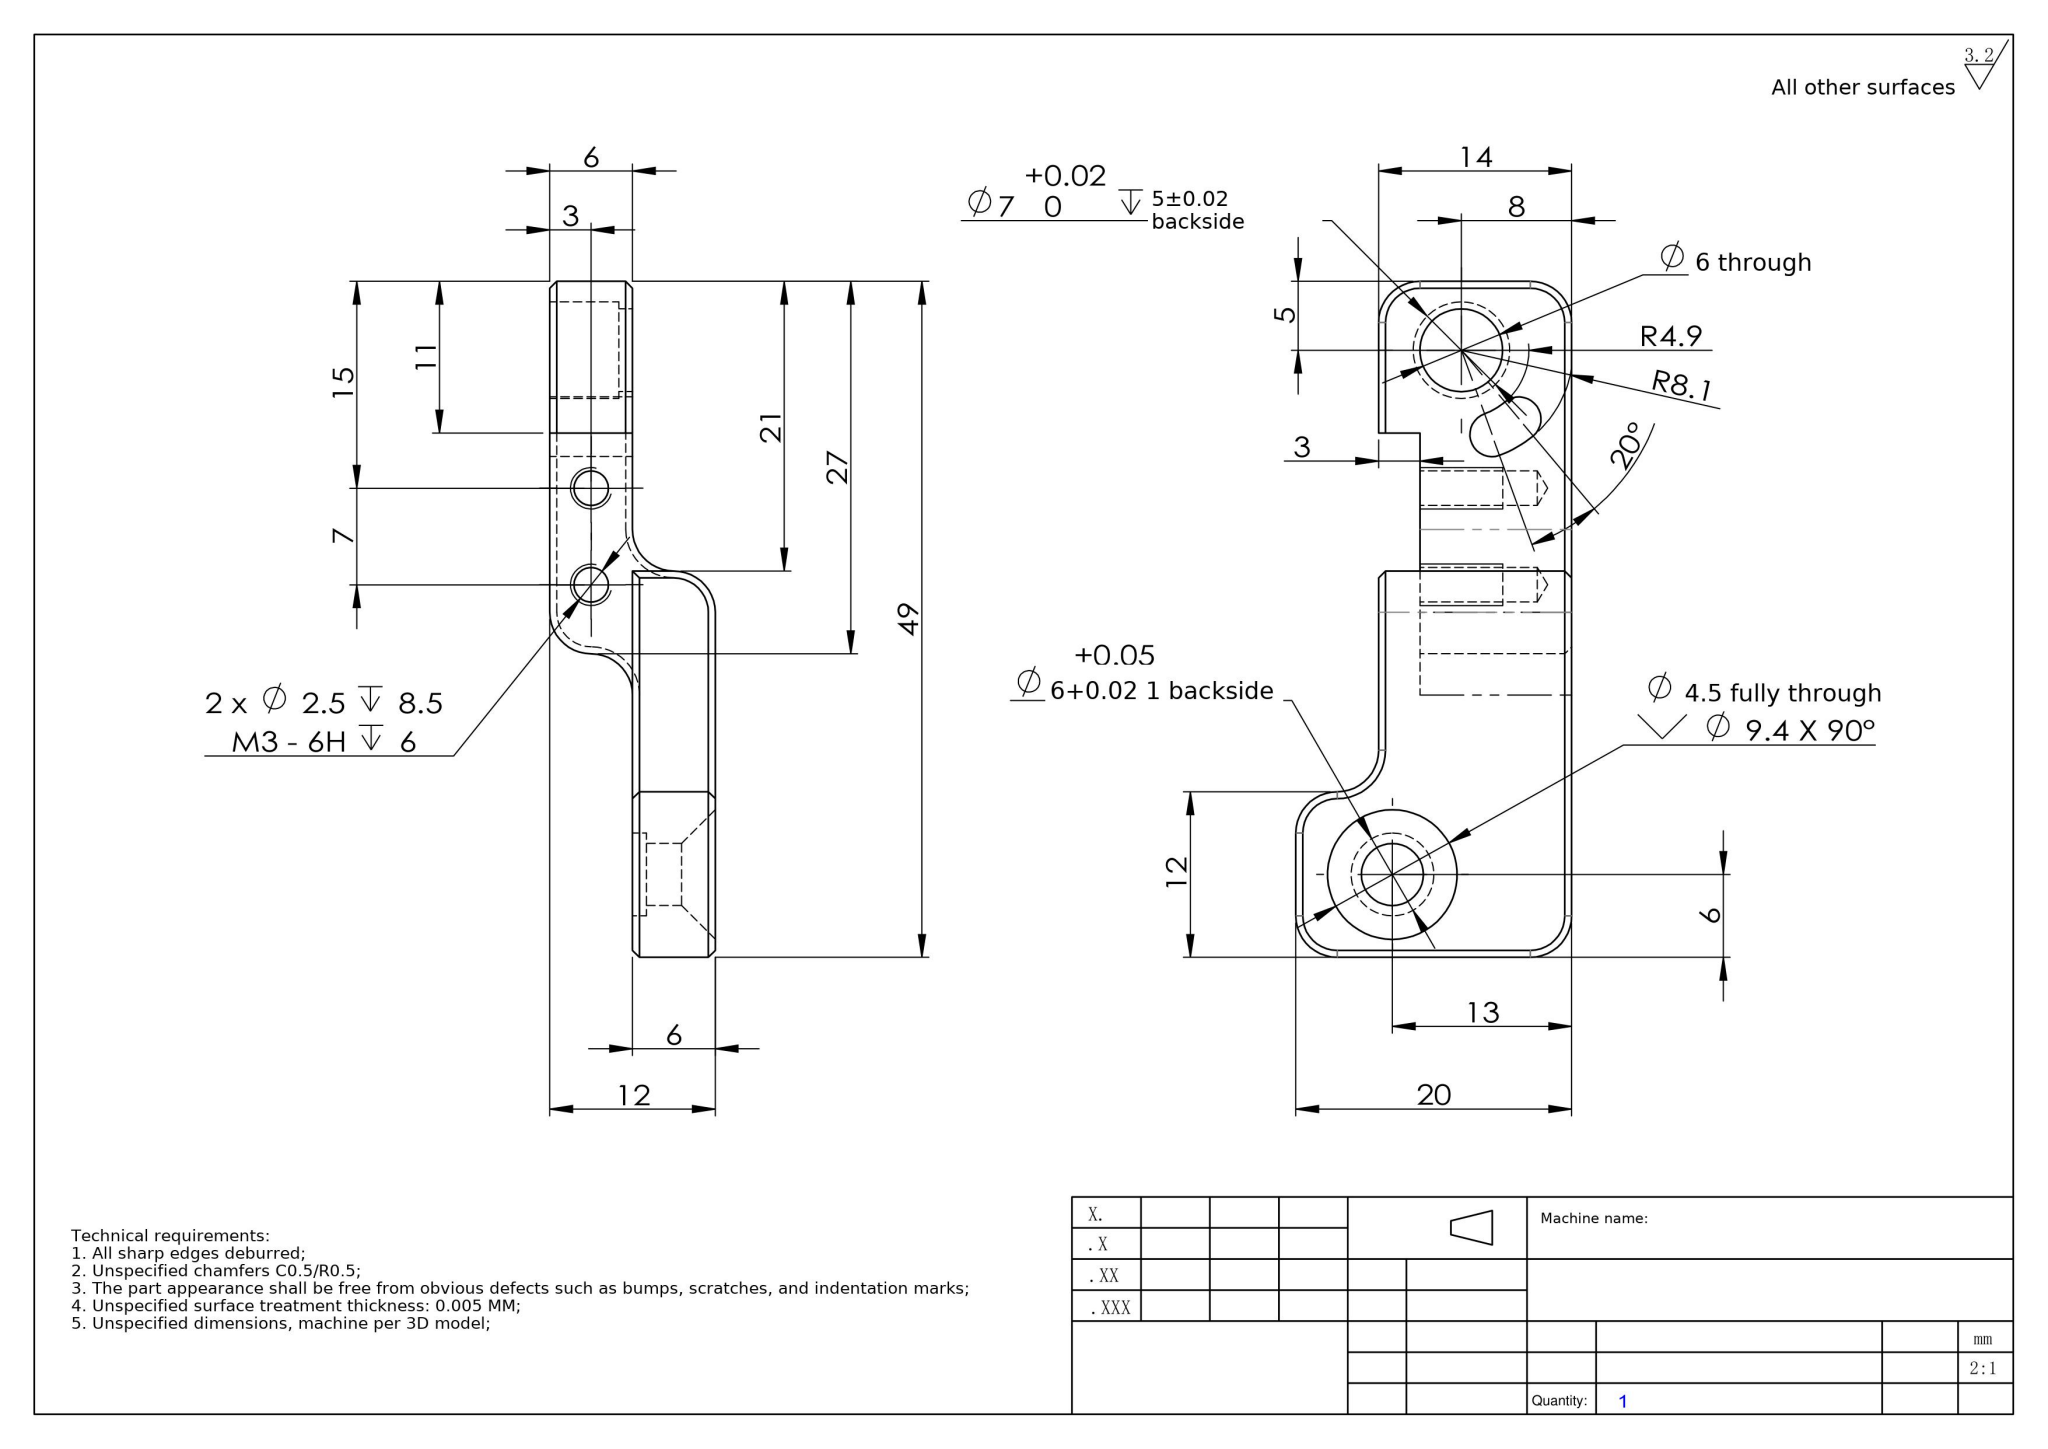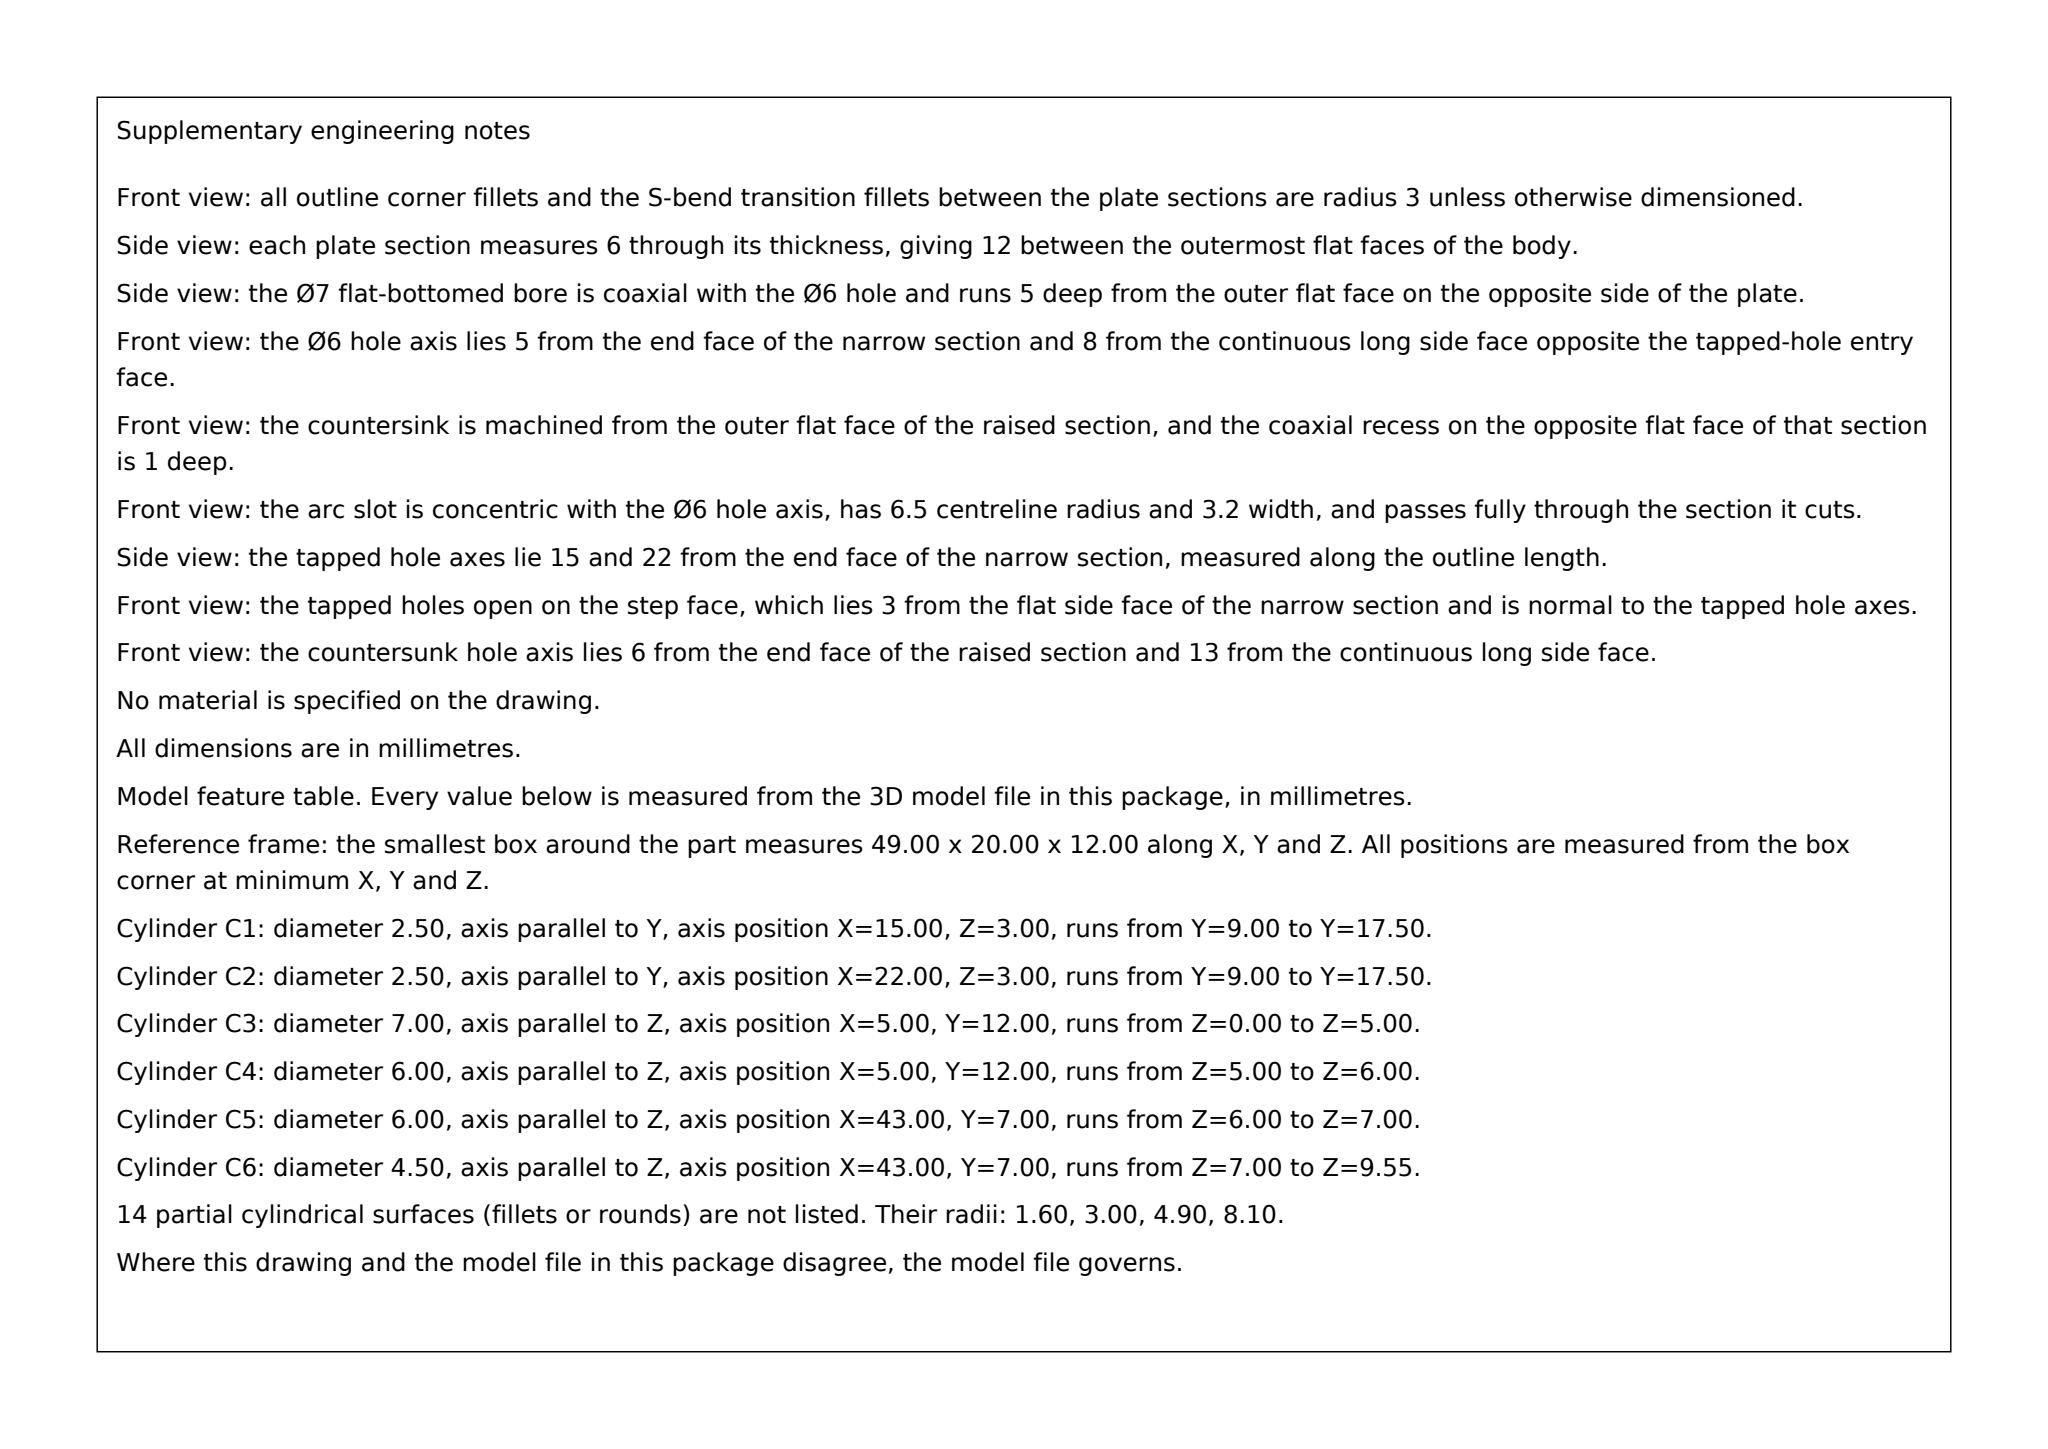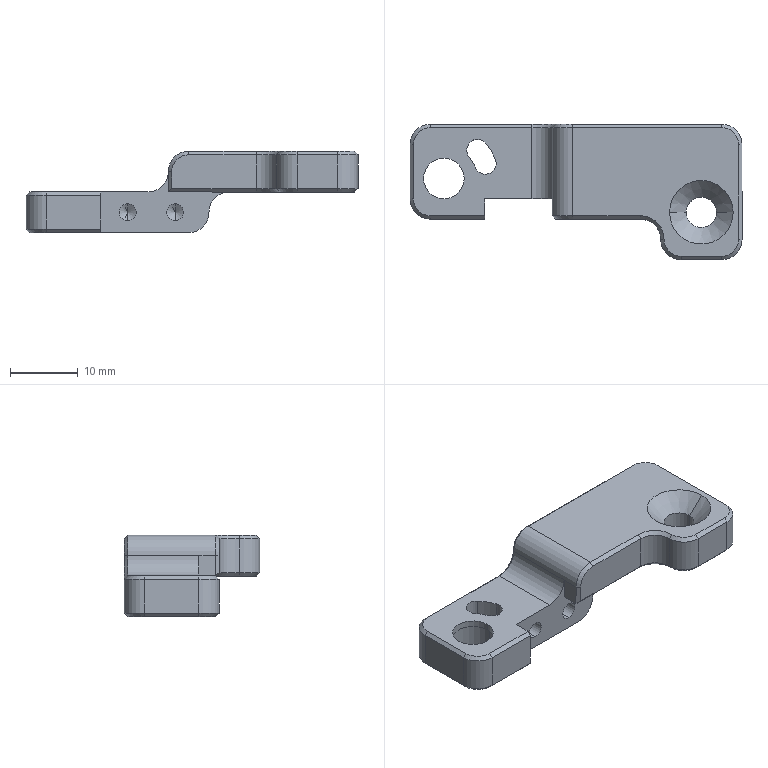Part | SolidWorks | mm | 1 solid | 80 faces | box 49 x 20 x 12 mm | volume 4117 mm3 | plane 30 | cylinder 27 | cone 23 | commonest cylinder face diameters 6 x14 2.5 x4 3.2 x3 4.5 x2 7 x2 9.8 x1 16.2 x1